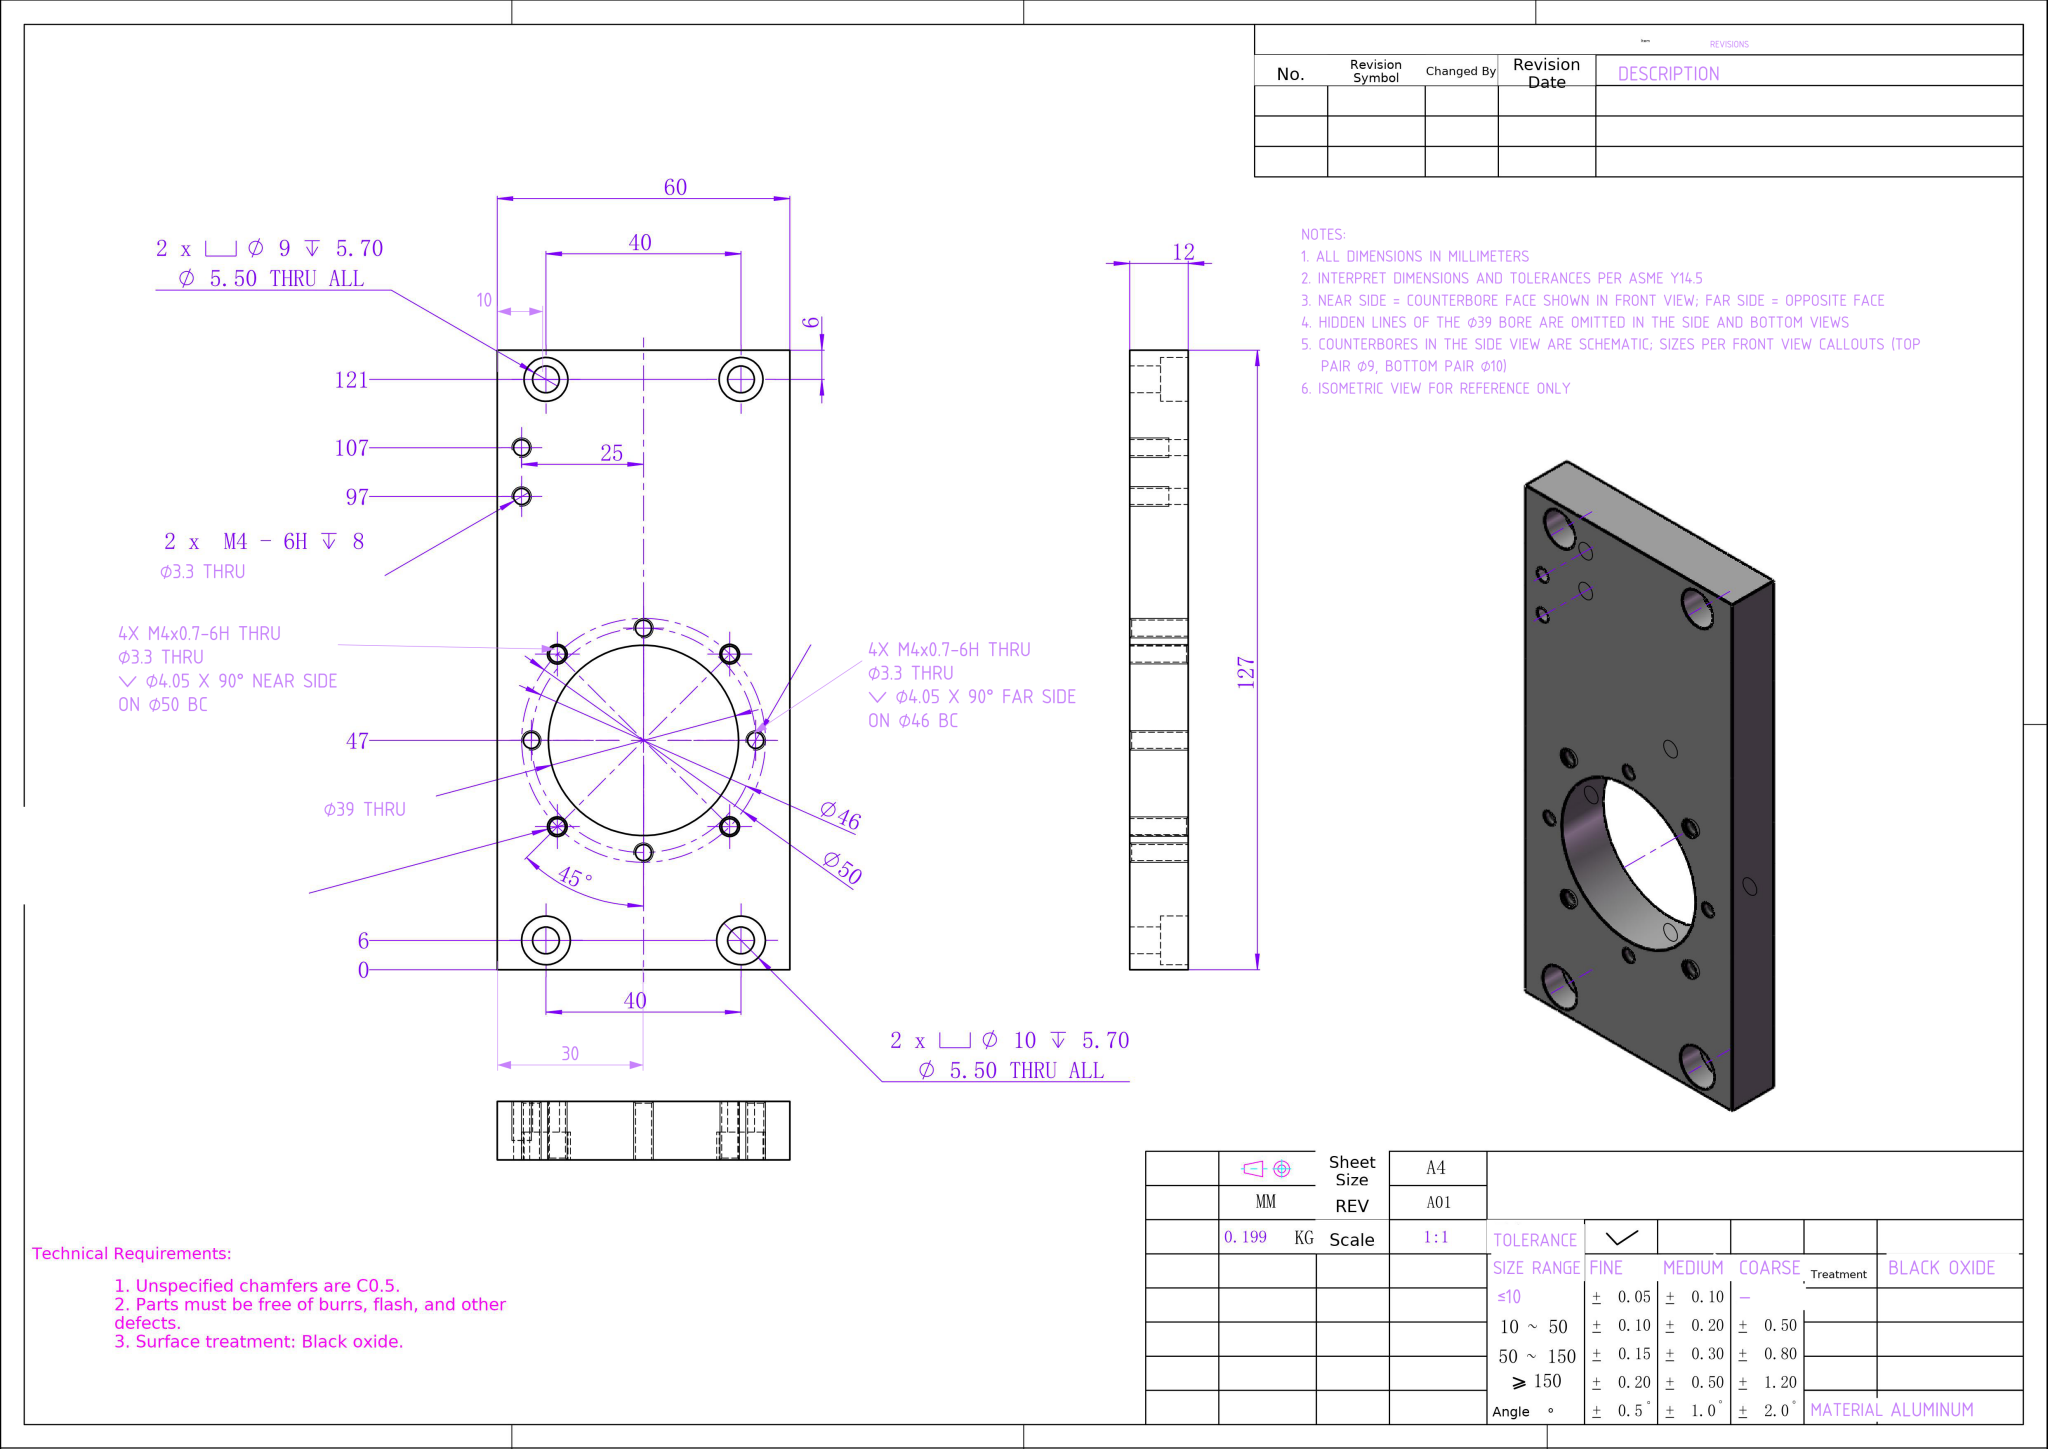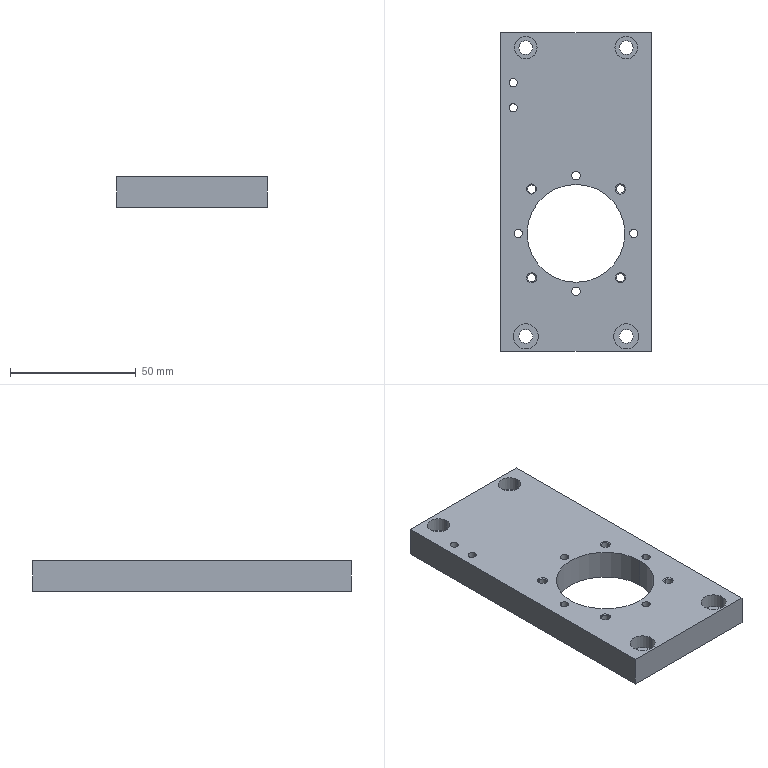Part | NX | mm | 1 solid | 64 faces | box 60 x 127 x 12 mm | volume 73853 mm3 | cylinder 38 | cone 16 | plane 10 | commonest cylinder face diameters 3.3 x20 5.5 x8 10 x4 9 x4 39 x2